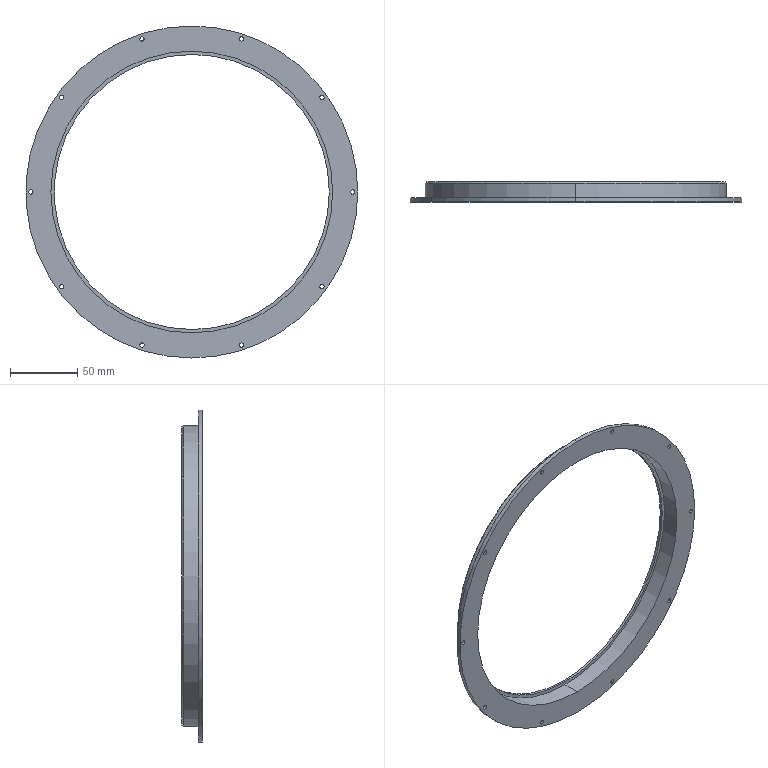CAM job | Mastercam | mm | 1 operations | part box 247.5 x 15 x 247.5
1. Drill/Counterbore | 7 - 4 倒角刀